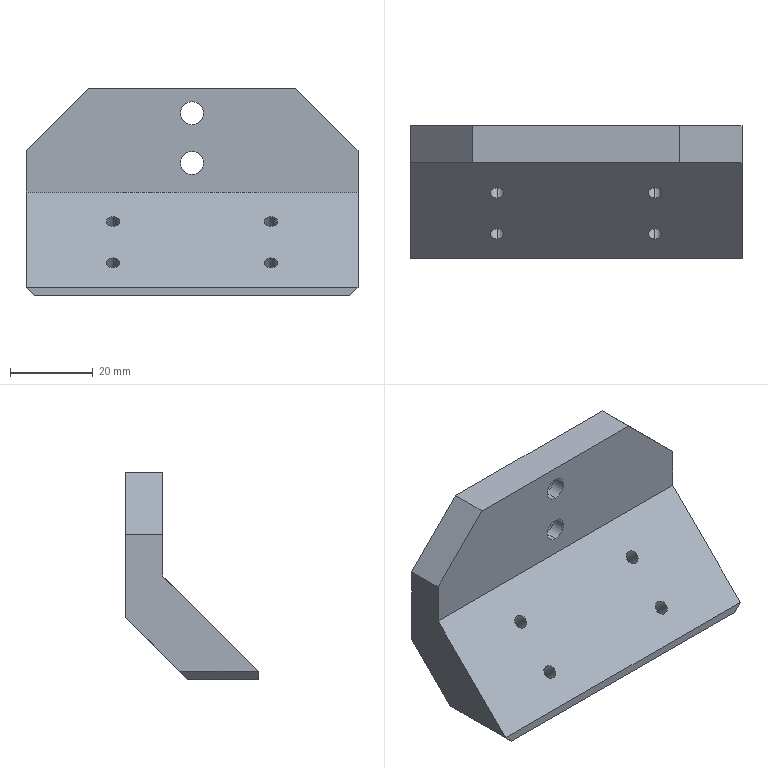Component | SolidWorks | ClampingArm2-1_A26-1 | 1 solid | 39 faces | box 80 x 32.02 x 50 mm | volume 48336 mm3 | cylinder 16 | plane 15 | cone 8 | commonest cylinder face diameters 3.3 x8 10 x4 5.5 x4 | material S45C
build123d program:
from build123d import *

# Parameters (mm, degrees)
SKETCH1_W                                          = 50
SKETCH1_H                                          = 60
BOSS_EXTRUDE1_DEPTH                                = 40
SKETCH2_OUTSIDE_W                                  = 74.36
SKETCH2_OUTSIDE_H                                  = 84.36
CUT_EXTRUDE1_DEPTH                                 = 90.022
HOLE_SIZE_ACCORDING_TO_TYPE_1_OF_HEXAG_D           = 5.5
HOLE_SIZE_ACCORDING_TO_TYPE_1_OF_HEXAG_CBORE_D     = 10
HOLE_SIZE_ACCORDING_TO_TYPE_1_OF_HEXAG_CBORE_DEPTH = 5.7
CHAMFER1_SIZE                                      = 2
CHAMFER2_SIZE                                      = 15
CHAMFER3_SIZE                                      = 15
M4_TAPPED_HOLE1_D                                  = 3.3
M4_TAPPED_HOLE1_DEPTH                              = 10.1
M4_TAPPED_HOLE1_TIP                                = 0.9914


with BuildPart() as part:
    # Sketch1 → Boss-Extrude1 (new, symmetric)
    with BuildSketch(Plane(origin=(0, 0, 0), x_dir=(0, 0, -1), z_dir=(1, 0, 0))):
        Rectangle(SKETCH1_W, SKETCH1_H)
    extrude(amount=BOSS_EXTRUDE1_DEPTH, both=True)

    # Sketch2 outside → Cut-Extrude1 (cut, through all)
    with BuildSketch(Plane(origin=(40, 0, 0), x_dir=(0, 0, -1), z_dir=(1, 0, 0))):
        Rectangle(SKETCH2_OUTSIDE_W, SKETCH2_OUTSIDE_H)
        Polygon((25, 21), (0, 21), (-23, -2), (-25, -2), (-25, 30), (25, 30), align=None, mode=Mode.SUBTRACT)
    extrude(amount=-CUT_EXTRUDE1_DEPTH, mode=Mode.SUBTRACT)

    # Hole Size _According to_ Type 1 of Hexag (through all)
    with Locations(Plane(origin=(0, 30, 0), x_dir=(1, 0, 0), z_dir=(0, 1, 0))):
        with Locations((0, 19), (0, 7)):
            CounterBoreHole(HOLE_SIZE_ACCORDING_TO_TYPE_1_OF_HEXAG_D / 2, HOLE_SIZE_ACCORDING_TO_TYPE_1_OF_HEXAG_CBORE_D / 2, HOLE_SIZE_ACCORDING_TO_TYPE_1_OF_HEXAG_CBORE_DEPTH)

    # Chamfer1
    chamfer1_edges = [part.edges().sort_by_distance(p)[0] for p in [
        (-40, 14, 25),
        (40, 14, 25),
    ]]
    chamfer(chamfer1_edges, length=CHAMFER1_SIZE)

    # Chamfer2
    chamfer2_edges = [part.edges().sort_by_distance(p)[0] for p in [
        (0, 30, 25),
    ]]
    chamfer(chamfer2_edges, length=CHAMFER2_SIZE)

    # Chamfer3
    chamfer3_edges = [part.edges().sort_by_distance(p)[0] for p in [
        (-40, 25.5, -25),
        (40, 25.5, -25),
    ]]
    chamfer(chamfer3_edges, length=CHAMFER3_SIZE)

    # M4 Tapped Hole1
    with Locations(Plane(origin=(0, 10.5, 10.5), x_dir=(-1, 0, 0), z_dir=(0, -0.7071, -0.7071))):
        with Locations((-19, -9.272), (-19, 4.728), (19, 4.728), (19, -9.272)):
            Hole(M4_TAPPED_HOLE1_D / 2, depth=M4_TAPPED_HOLE1_DEPTH)
            with Locations((0, 0, -(M4_TAPPED_HOLE1_DEPTH + M4_TAPPED_HOLE1_TIP / 2))):  # 118° drill point
                Cone(0, M4_TAPPED_HOLE1_D / 2, M4_TAPPED_HOLE1_TIP, mode=Mode.SUBTRACT)


solid = part.part

# Placed as in the assembly
solid = solid.moved(Location((-43.051, 45.001, -157.493), (179.981, 0, -180)))